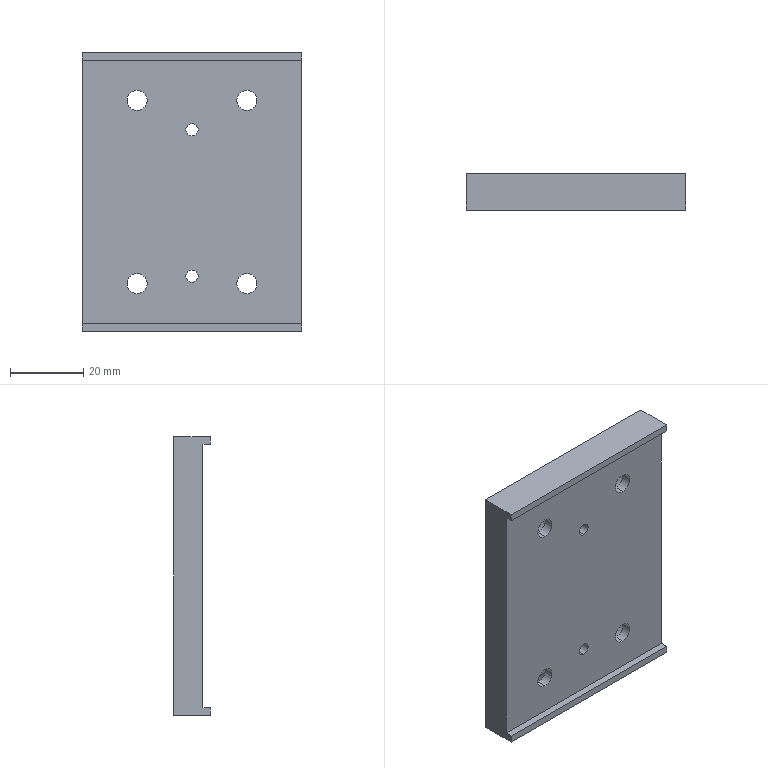Part | SolidWorks | mm | 1 solid | 43 faces | box 60 x 10 x 76 mm | volume 34729 mm3 | cylinder 24 | plane 14 | cone 5 | commonest cylinder face diameters 3.3 x8 10 x8 5.5 x8
Drawing notes:
RIGHT VIEW: 74.00 FROM BOTTOM EDGE (0) TO STEP FACE | from the solid: axis_planes z=0.0 and z=74.0; top face z=76.0 (bbox Z 76.001)
build123d program:
from build123d import *

# Parameters (mm, degrees)
SKETCH1_W                                       = 60
SKETCH1_H                                       = 76
BOSS_EXTRUDE1_DEPTH                             = 10
SKETCH2_W                                       = 60
SKETCH2_H                                       = 72
CUT_EXTRUDE1_DEPTH                              = 2
M4_TAPPED_HOLE1_D                               = 3.3
M5_HEX_SOCKET_HEAD_CAP_SCREW_CBORE1_D           = 5.5
M5_HEX_SOCKET_HEAD_CAP_SCREW_CBORE1_CBORE_D     = 10
M5_HEX_SOCKET_HEAD_CAP_SCREW_CBORE1_CBORE_DEPTH = 5.4
M4_TAPPED_HOLE2_D                               = 3.3
M4_TAPPED_HOLE2_DEPTH                           = 10.1
M4_TAPPED_HOLE2_TIP                             = 0.9914


with BuildPart() as part:
    # Sketch1 → Boss-Extrude1 (new body)
    with BuildSketch(Plane(origin=(0, 0, 0), x_dir=(1, 0, 0), z_dir=(0, 1, 0))):
        with Locations((30, 38)):
            Rectangle(SKETCH1_W, SKETCH1_H)
    extrude(amount=BOSS_EXTRUDE1_DEPTH)

    # Sketch2 → Cut-Extrude1 (cut)
    with BuildSketch(Plane.XZ):
        with Locations((30, -38)):
            Rectangle(SKETCH2_W, SKETCH2_H)
    extrude(amount=-CUT_EXTRUDE1_DEPTH, mode=Mode.SUBTRACT)

    # M4 Tapped Hole1 (through all)
    with Locations(Plane(origin=(0, 10, 0), x_dir=(1, 0, 0), z_dir=(0, 1, 0))):
        with Locations((30, 61), (30, 21)):
            Hole(M4_TAPPED_HOLE1_D / 2)

    # M5 Hex Socket Head Cap Screw CBORE1 (through all)
    with Locations(Plane(origin=(0, 10, 0), x_dir=(1, 0, 0), z_dir=(0, 1, 0))):
        with Locations((15, 13), (45, 13), (45, 63), (15, 63)):
            CounterBoreHole(M5_HEX_SOCKET_HEAD_CAP_SCREW_CBORE1_D / 2, M5_HEX_SOCKET_HEAD_CAP_SCREW_CBORE1_CBORE_D / 2, M5_HEX_SOCKET_HEAD_CAP_SCREW_CBORE1_CBORE_DEPTH)

    # M4 Tapped Hole2
    with Locations(Plane(origin=(0, 0, -76), x_dir=(-1, 0, 0), z_dir=(0, 0, -1))):
        with Locations((-17.5, 6), (-42.5, 6)):
            Hole(M4_TAPPED_HOLE2_D / 2, depth=M4_TAPPED_HOLE2_DEPTH)
            with Locations((0, 0, -(M4_TAPPED_HOLE2_DEPTH + M4_TAPPED_HOLE2_TIP / 2))):  # 118° drill point
                Cone(0, M4_TAPPED_HOLE2_D / 2, M4_TAPPED_HOLE2_TIP, mode=Mode.SUBTRACT)


solid = part.part